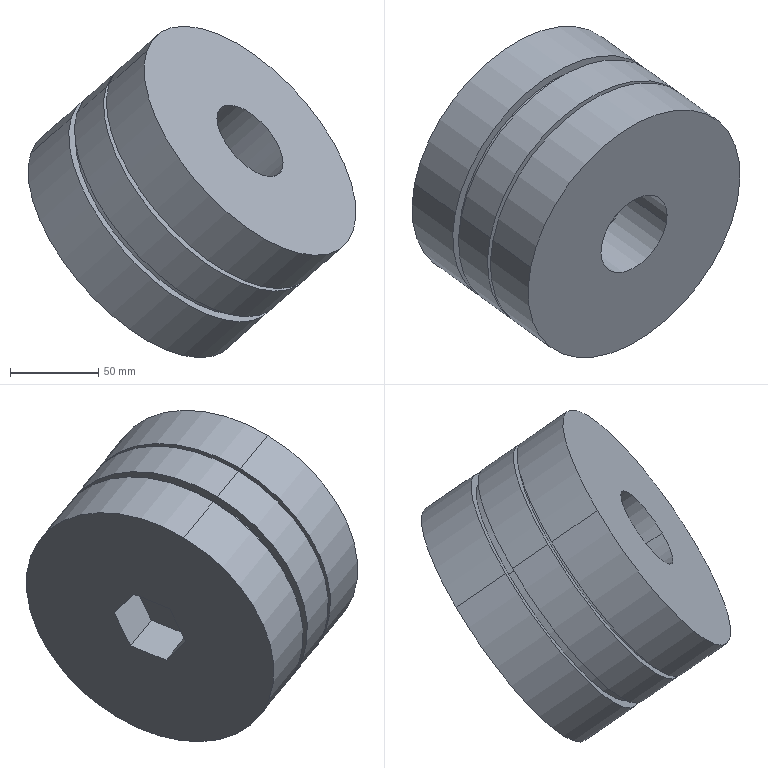Component | SolidWorks | FrictionWasher-1 | 1 solid | 29 faces | box 186.23 x 188.32 x 188.31 mm | volume 1876724 mm3 | plane 15 | cylinder 14 | commonest cylinder face diameters 160 x6 150 x4 50 x2 25 x2 | material Copper
STEP:
#1=CARTESIAN_POINT('',(0.3939,-67.745,7.065));
#2=VERTEX_POINT('',#1);
#3=CARTESIAN_POINT('',(-4.23,-69.254,11.068));
#4=VERTEX_POINT('',#3);
#5=CARTESIAN_POINT('',(-1.918,-68.5,9.067));
#6=DIRECTION('',(0.6592,-0.4763,0.5818));
#7=DIRECTION('',(0.734,0.2396,-0.6355));
#8=AXIS2_PLACEMENT_3D('',#5,#6,#7);
#9=CIRCLE('',#8,3.15);
#10=EDGE_CURVE('',#2,#4,#9,.T.);
#11=ORIENTED_EDGE('',*,*,#10,.F.);
#12=CARTESIAN_POINT('',(-0.4496,-67.136,6.321));
#13=VERTEX_POINT('',#12);
#14=CARTESIAN_POINT('',(0.3939,-67.745,7.065));
#15=DIRECTION('',(-0.6592,0.4763,-0.5818));
#16=VECTOR('',#15,39.37);
#17=LINE('',#14,#16);
#18=EDGE_CURVE('',#2,#13,#17,.T.);
#19=ORIENTED_EDGE('',*,*,#18,.T.);
#20=CARTESIAN_POINT('',(-5.073,-68.645,10.324));
#21=VERTEX_POINT('',#20);
#22=CARTESIAN_POINT('',(-2.761,-67.89,8.322));
#23=DIRECTION('',(-0.6592,0.4763,-0.5818));
#24=DIRECTION('',(-0.734,-0.2396,0.6355));
#25=AXIS2_PLACEMENT_3D('',#22,#23,#24);
#26=CIRCLE('',#25,3.15);
#27=EDGE_CURVE('',#21,#13,#26,.T.);
#28=ORIENTED_EDGE('',*,*,#27,.F.);
#29=CARTESIAN_POINT('',(-4.23,-69.254,11.068));
#30=DIRECTION('',(-0.6592,0.4763,-0.5818));
#31=VECTOR('',#30,39.37);
#32=LINE('',#29,#31);
#33=EDGE_CURVE('',#4,#21,#32,.T.);
#34=ORIENTED_EDGE('',*,*,#33,.F.);
#35=EDGE_LOOP('',(#11,#19,#28,#34));
#36=FACE_OUTER_BOUND('',#35,.T.);
#37=CARTESIAN_POINT('',(-1.918,-68.5,9.067));
#38=DIRECTION('',(-0.6592,0.4763,-0.5818));
#39=DIRECTION('',(-0.734,-0.2396,0.6355));
#40=AXIS2_PLACEMENT_3D('',#37,#38,#39);
#41=CYLINDRICAL_SURFACE('',#40,3.15);
#42=ADVANCED_FACE('',(#36),#41,.T.);
#43=CARTESIAN_POINT('',(-2.64,-68.736,9.692));
#44=VERTEX_POINT('',#43);
#45=CARTESIAN_POINT('',(-1.195,-68.264,8.441));
#46=VERTEX_POINT('',#45);
#47=CARTESIAN_POINT('',(-1.918,-68.5,9.067));
#48=DIRECTION('',(0.6592,-0.4763,0.5818));
#49=DIRECTION('',(0.734,0.2396,-0.6355));
#50=AXIS2_PLACEMENT_3D('',#47,#48,#49);
#51=CIRCLE('',#50,0.9843);
#52=EDGE_CURVE('',#44,#46,#51,.T.);
#53=ORIENTED_EDGE('',*,*,#52,.T.);
#54=CARTESIAN_POINT('',(-2.104,-67.608,7.64));
#55=VERTEX_POINT('',#54);
#56=CARTESIAN_POINT('',(-1.195,-68.264,8.441));
#57=DIRECTION('',(-0.6592,0.4763,-0.5818));
#58=VECTOR('',#57,39.37);
#59=LINE('',#56,#58);
#60=EDGE_CURVE('',#46,#55,#59,.T.);
#61=ORIENTED_EDGE('',*,*,#60,.T.);
#62=CARTESIAN_POINT('',(-3.549,-68.079,8.891));
#63=VERTEX_POINT('',#62);
#64=CARTESIAN_POINT('',(-2.826,-67.843,8.265));
#65=DIRECTION('',(0.6592,-0.4763,0.5818));
#66=DIRECTION('',(0.734,0.2396,-0.6355));
#67=AXIS2_PLACEMENT_3D('',#64,#65,#66);
#68=CIRCLE('',#67,0.9843);
#69=EDGE_CURVE('',#63,#55,#68,.T.);
#70=ORIENTED_EDGE('',*,*,#69,.F.);
#71=CARTESIAN_POINT('',(-2.64,-68.736,9.692));
#72=DIRECTION('',(-0.6592,0.4763,-0.5818));
#73=VECTOR('',#72,39.37);
#74=LINE('',#71,#73);
#75=EDGE_CURVE('',#44,#63,#74,.T.);
#76=ORIENTED_EDGE('',*,*,#75,.F.);
#77=EDGE_LOOP('',(#53,#61,#70,#76));
#78=FACE_OUTER_BOUND('',#77,.T.);
#79=CARTESIAN_POINT('',(-1.918,-68.5,9.067));
#80=DIRECTION('',(-0.6592,0.4763,-0.5818));
#81=DIRECTION('',(-0.734,-0.2396,0.6355));
#82=AXIS2_PLACEMENT_3D('',#79,#80,#81);
#83=CYLINDRICAL_SURFACE('',#82,0.9843);
#84=ADVANCED_FACE('',(#78),#83,.F.);
#85=CARTESIAN_POINT('',(-3.187,-67.961,8.578));
#86=VERTEX_POINT('',#85);
#87=CARTESIAN_POINT('',(-2.465,-67.726,7.952));
#88=VERTEX_POINT('',#87);
#89=CARTESIAN_POINT('',(-2.826,-67.843,8.265));
#90=DIRECTION('',(0.6592,-0.4763,0.5818));
#91=DIRECTION('',(0.734,0.2396,-0.6355));
#92=AXIS2_PLACEMENT_3D('',#89,#90,#91);
#93=CIRCLE('',#92,0.4921);
#94=EDGE_CURVE('',#86,#88,#93,.T.);
#95=ORIENTED_EDGE('',*,*,#94,.T.);
#96=CARTESIAN_POINT('',(-3.114,-67.257,7.38));
#97=VERTEX_POINT('',#96);
#98=CARTESIAN_POINT('',(-2.465,-67.726,7.952));
#99=DIRECTION('',(-0.6592,0.4763,-0.5818));
#100=VECTOR('',#99,39.37);
#101=LINE('',#98,#100);
#102=EDGE_CURVE('',#88,#97,#101,.T.);
#103=ORIENTED_EDGE('',*,*,#102,.T.);
#104=CARTESIAN_POINT('',(-3.836,-67.493,8.005));
#105=VERTEX_POINT('',#104);
#106=CARTESIAN_POINT('',(-3.475,-67.375,7.692));
#107=DIRECTION('',(0.6592,-0.4763,0.5818));
#108=DIRECTION('',(0.734,0.2396,-0.6355));
#109=AXIS2_PLACEMENT_3D('',#106,#107,#108);
#110=CIRCLE('',#109,0.4921);
#111=EDGE_CURVE('',#105,#97,#110,.T.);
#112=ORIENTED_EDGE('',*,*,#111,.F.);
#113=CARTESIAN_POINT('',(-3.187,-67.961,8.578));
#114=DIRECTION('',(-0.6592,0.4763,-0.5818));
#115=VECTOR('',#114,39.37);
#116=LINE('',#113,#115);
#117=EDGE_CURVE('',#86,#105,#116,.T.);
#118=ORIENTED_EDGE('',*,*,#117,.F.);
#119=EDGE_LOOP('',(#95,#103,#112,#118));
#120=FACE_OUTER_BOUND('',#119,.T.);
#121=CARTESIAN_POINT('',(-2.826,-67.843,8.265));
#122=DIRECTION('',(-0.6592,0.4763,-0.5818));
#123=DIRECTION('',(-0.734,-0.2396,0.6355));
#124=AXIS2_PLACEMENT_3D('',#121,#122,#123);
#125=CYLINDRICAL_SURFACE('',#124,0.4921);
#126=ADVANCED_FACE('',(#120),#125,.F.);
#127=CARTESIAN_POINT('',(-4.929,-68.598,10.199));
#128=VERTEX_POINT('',#127);
#129=CARTESIAN_POINT('',(-0.5941,-67.183,6.446));
#130=VERTEX_POINT('',#129);
#131=CARTESIAN_POINT('',(-2.761,-67.89,8.322));
#132=DIRECTION('',(-0.6592,0.4763,-0.5818));
#133=DIRECTION('',(-0.1633,-0.846,-0.5075));
#134=AXIS2_PLACEMENT_3D('',#131,#132,#133);
#135=CIRCLE('',#134,2.953);
#136=EDGE_CURVE('',#128,#130,#135,.T.);
#137=ORIENTED_EDGE('',*,*,#136,.T.);
#138=CARTESIAN_POINT('',(-0.659,-67.136,6.389));
#139=VERTEX_POINT('',#138);
#140=CARTESIAN_POINT('',(-0.5941,-67.183,6.446));
#141=DIRECTION('',(-0.6592,0.4763,-0.5818));
#142=VECTOR('',#141,39.37);
#143=LINE('',#140,#142);
#144=EDGE_CURVE('',#130,#139,#143,.T.);
#145=ORIENTED_EDGE('',*,*,#144,.T.);
#146=CARTESIAN_POINT('',(-4.994,-68.551,10.142));
#147=VERTEX_POINT('',#146);
#148=CARTESIAN_POINT('',(-2.826,-67.843,8.265));
#149=DIRECTION('',(-0.6592,0.4763,-0.5818));
#150=DIRECTION('',(-0.1633,-0.846,-0.5075));
#151=AXIS2_PLACEMENT_3D('',#148,#149,#150);
#152=CIRCLE('',#151,2.953);
#153=EDGE_CURVE('',#147,#139,#152,.T.);
#154=ORIENTED_EDGE('',*,*,#153,.F.);
#155=CARTESIAN_POINT('',(-4.929,-68.598,10.199));
#156=DIRECTION('',(-0.6592,0.4763,-0.5818));
#157=VECTOR('',#156,39.37);
#158=LINE('',#155,#157);
#159=EDGE_CURVE('',#128,#147,#158,.T.);
#160=ORIENTED_EDGE('',*,*,#159,.F.);
#161=EDGE_LOOP('',(#137,#145,#154,#160));
#162=FACE_OUTER_BOUND('',#161,.T.);
#163=CARTESIAN_POINT('',(-2.761,-67.89,8.322));
#164=DIRECTION('',(-0.6592,0.4763,-0.5818));
#165=DIRECTION('',(-0.734,-0.2396,0.6355));
#166=AXIS2_PLACEMENT_3D('',#163,#164,#165);
#167=CYLINDRICAL_SURFACE('',#166,2.953);
#168=ADVANCED_FACE('',(#162),#167,.T.);
#169=CARTESIAN_POINT('',(-5.917,-68.035,9.58));
#170=VERTEX_POINT('',#169);
#171=CARTESIAN_POINT('',(-1.293,-66.526,5.576));
#172=VERTEX_POINT('',#171);
#173=CARTESIAN_POINT('',(-3.605,-67.281,7.578));
#174=DIRECTION('',(-0.6592,0.4763,-0.5818));
#175=DIRECTION('',(-0.734,-0.2396,0.6355));
#176=AXIS2_PLACEMENT_3D('',#173,#174,#175);
#177=CIRCLE('',#176,3.15);
#178=EDGE_CURVE('',#170,#172,#177,.T.);
#179=ORIENTED_EDGE('',*,*,#178,.T.);
#180=CARTESIAN_POINT('',(-2.201,-65.87,4.775));
#181=VERTEX_POINT('',#180);
#182=CARTESIAN_POINT('',(0.3939,-67.745,7.065));
#183=DIRECTION('',(-0.6592,0.4763,-0.5818));
#184=VECTOR('',#183,39.37);
#185=LINE('',#182,#184);
#186=EDGE_CURVE('',#172,#181,#185,.T.);
#187=ORIENTED_EDGE('',*,*,#186,.T.);
#188=CARTESIAN_POINT('',(-6.825,-67.379,8.778));
#189=VERTEX_POINT('',#188);
#190=CARTESIAN_POINT('',(-4.513,-66.625,6.776));
#191=DIRECTION('',(0.6592,-0.4763,0.5818));
#192=DIRECTION('',(0.734,0.2396,-0.6355));
#193=AXIS2_PLACEMENT_3D('',#190,#191,#192);
#194=CIRCLE('',#193,3.15);
#195=EDGE_CURVE('',#181,#189,#194,.T.);
#196=ORIENTED_EDGE('',*,*,#195,.T.);
#197=CARTESIAN_POINT('',(-4.23,-69.254,11.068));
#198=DIRECTION('',(-0.6592,0.4763,-0.5818));
#199=VECTOR('',#198,39.37);
#200=LINE('',#197,#199);
#201=EDGE_CURVE('',#170,#189,#200,.T.);
#202=ORIENTED_EDGE('',*,*,#201,.F.);
#203=EDGE_LOOP('',(#179,#187,#196,#202));
#204=FACE_OUTER_BOUND('',#203,.T.);
#205=CARTESIAN_POINT('',(-1.918,-68.5,9.067));
#206=DIRECTION('',(-0.6592,0.4763,-0.5818));
#207=DIRECTION('',(-0.734,-0.2396,0.6355));
#208=AXIS2_PLACEMENT_3D('',#205,#206,#207);
#209=CYLINDRICAL_SURFACE('',#208,3.15);
#210=ADVANCED_FACE('',(#204),#209,.T.);
#211=CARTESIAN_POINT('',(-5.642,-68.082,9.569));
#212=VERTEX_POINT('',#211);
#213=CARTESIAN_POINT('',(-1.308,-66.667,5.816));
#214=VERTEX_POINT('',#213);
#215=CARTESIAN_POINT('',(-3.475,-67.375,7.692));
#216=DIRECTION('',(-0.6592,0.4763,-0.5818));
#217=DIRECTION('',(-0.1633,-0.846,-0.5075));
#218=AXIS2_PLACEMENT_3D('',#215,#216,#217);
#219=CIRCLE('',#218,2.953);
#220=EDGE_CURVE('',#212,#214,#219,.T.);
#221=ORIENTED_EDGE('',*,*,#220,.T.);
#222=CARTESIAN_POINT('',(-1.438,-66.574,5.701));
#223=VERTEX_POINT('',#222);
#224=CARTESIAN_POINT('',(-1.308,-66.667,5.816));
#225=DIRECTION('',(-0.6592,0.4763,-0.5818));
#226=VECTOR('',#225,39.37);
#227=LINE('',#224,#226);
#228=EDGE_CURVE('',#214,#223,#227,.T.);
#229=ORIENTED_EDGE('',*,*,#228,.T.);
#230=CARTESIAN_POINT('',(-5.772,-67.988,9.454));
#231=VERTEX_POINT('',#230);
#232=CARTESIAN_POINT('',(-3.605,-67.281,7.578));
#233=DIRECTION('',(-0.6592,0.4763,-0.5818));
#234=DIRECTION('',(-0.1633,-0.846,-0.5075));
#235=AXIS2_PLACEMENT_3D('',#232,#233,#234);
#236=CIRCLE('',#235,2.953);
#237=EDGE_CURVE('',#231,#223,#236,.T.);
#238=ORIENTED_EDGE('',*,*,#237,.F.);
#239=CARTESIAN_POINT('',(-5.642,-68.082,9.569));
#240=DIRECTION('',(-0.6592,0.4763,-0.5818));
#241=VECTOR('',#240,39.37);
#242=LINE('',#239,#241);
#243=EDGE_CURVE('',#212,#231,#242,.T.);
#244=ORIENTED_EDGE('',*,*,#243,.F.);
#245=EDGE_LOOP('',(#221,#229,#238,#244));
#246=FACE_OUTER_BOUND('',#245,.T.);
#247=CARTESIAN_POINT('',(-3.475,-67.375,7.692));
#248=DIRECTION('',(-0.6592,0.4763,-0.5818));
#249=DIRECTION('',(-0.734,-0.2396,0.6355));
#250=AXIS2_PLACEMENT_3D('',#247,#248,#249);
#251=CYLINDRICAL_SURFACE('',#250,2.953);
#252=ADVANCED_FACE('',(#246),#251,.T.);
#253=CARTESIAN_POINT('',(-5.138,-68.598,10.267));
#254=VERTEX_POINT('',#253);
#255=CARTESIAN_POINT('',(-0.5145,-67.089,6.264));
#256=VERTEX_POINT('',#255);
#257=CARTESIAN_POINT('',(-2.826,-67.843,8.265));
#258=DIRECTION('',(-0.6592,0.4763,-0.5818));
#259=DIRECTION('',(-0.734,-0.2396,0.6355));
#260=AXIS2_PLACEMENT_3D('',#257,#258,#259);
#261=CIRCLE('',#260,3.15);
#262=EDGE_CURVE('',#254,#256,#261,.T.);
#263=ORIENTED_EDGE('',*,*,#262,.T.);
#264=CARTESIAN_POINT('',(-1.163,-66.62,5.691));
#265=VERTEX_POINT('',#264);
#266=CARTESIAN_POINT('',(0.3939,-67.745,7.065));
#267=DIRECTION('',(-0.6592,0.4763,-0.5818));
#268=VECTOR('',#267,39.37);
#269=LINE('',#266,#268);
#270=EDGE_CURVE('',#256,#265,#269,.T.);
#271=ORIENTED_EDGE('',*,*,#270,.T.);
#272=CARTESIAN_POINT('',(-5.787,-68.129,9.694));
#273=VERTEX_POINT('',#272);
#274=CARTESIAN_POINT('',(-3.475,-67.375,7.692));
#275=DIRECTION('',(-0.6592,0.4763,-0.5818));
#276=DIRECTION('',(-0.734,-0.2396,0.6355));
#277=AXIS2_PLACEMENT_3D('',#274,#275,#276);
#278=CIRCLE('',#277,3.15);
#279=EDGE_CURVE('',#273,#265,#278,.T.);
#280=ORIENTED_EDGE('',*,*,#279,.F.);
#281=CARTESIAN_POINT('',(-4.23,-69.254,11.068));
#282=DIRECTION('',(-0.6592,0.4763,-0.5818));
#283=VECTOR('',#282,39.37);
#284=LINE('',#281,#283);
#285=EDGE_CURVE('',#254,#273,#284,.T.);
#286=ORIENTED_EDGE('',*,*,#285,.F.);
#287=EDGE_LOOP('',(#263,#271,#280,#286));
#288=FACE_OUTER_BOUND('',#287,.T.);
#289=CARTESIAN_POINT('',(-1.918,-68.5,9.067));
#290=DIRECTION('',(-0.6592,0.4763,-0.5818));
#291=DIRECTION('',(-0.734,-0.2396,0.6355));
#292=AXIS2_PLACEMENT_3D('',#289,#290,#291);
#293=CYLINDRICAL_SURFACE('',#292,3.15);
#294=ADVANCED_FACE('',(#288),#293,.T.);
#295=ORIENTED_EDGE('',*,*,#270,.F.);
#296=CARTESIAN_POINT('',(-2.826,-67.843,8.265));
#297=DIRECTION('',(-0.6592,0.4763,-0.5818));
#298=DIRECTION('',(-0.734,-0.2396,0.6355));
#299=AXIS2_PLACEMENT_3D('',#296,#297,#298);
#300=CIRCLE('',#299,3.15);
#301=EDGE_CURVE('',#256,#254,#300,.T.);
#302=ORIENTED_EDGE('',*,*,#301,.T.);
#303=ORIENTED_EDGE('',*,*,#285,.T.);
#304=CARTESIAN_POINT('',(-3.475,-67.375,7.692));
#305=DIRECTION('',(-0.6592,0.4763,-0.5818));
#306=DIRECTION('',(-0.734,-0.2396,0.6355));
#307=AXIS2_PLACEMENT_3D('',#304,#305,#306);
#308=CIRCLE('',#307,3.15);
#309=EDGE_CURVE('',#265,#273,#308,.T.);
#310=ORIENTED_EDGE('',*,*,#309,.F.);
#311=EDGE_LOOP('',(#295,#302,#303,#310));
#312=FACE_OUTER_BOUND('',#311,.T.);
#313=CARTESIAN_POINT('',(-1.918,-68.5,9.067));
#314=DIRECTION('',(-0.6592,0.4763,-0.5818));
#315=DIRECTION('',(-0.734,-0.2396,0.6355));
#316=AXIS2_PLACEMENT_3D('',#313,#314,#315);
#317=CYLINDRICAL_SURFACE('',#316,3.15);
#318=ADVANCED_FACE('',(#312),#317,.T.);
#319=ORIENTED_EDGE('',*,*,#220,.F.);
#320=CARTESIAN_POINT('',(-3.475,-67.375,7.692));
#321=DIRECTION('',(-0.6592,0.4763,-0.5818));
#322=DIRECTION('',(-0.1633,-0.846,-0.5075));
#323=AXIS2_PLACEMENT_3D('',#320,#321,#322);
#324=CIRCLE('',#323,2.953);
#325=EDGE_CURVE('',#214,#212,#324,.T.);
#326=ORIENTED_EDGE('',*,*,#325,.F.);
#327=EDGE_LOOP('',(#319,#326));
#328=FACE_BOUND('',#327,.T.);
#329=ORIENTED_EDGE('',*,*,#279,.T.);
#330=ORIENTED_EDGE('',*,*,#309,.T.);
#331=EDGE_LOOP('',(#329,#330));
#332=FACE_OUTER_BOUND('',#331,.T.);
#333=CARTESIAN_POINT('',(-3.475,-67.375,7.692));
#334=DIRECTION('',(-0.6592,0.4763,-0.5818));
#335=DIRECTION('',(-0.734,-0.2396,0.6355));
#336=AXIS2_PLACEMENT_3D('',#333,#334,#335);
#337=PLANE('',#336);
#338=ADVANCED_FACE('',(#328,#332),#337,.T.);
#339=ORIENTED_EDGE('',*,*,#237,.T.);
#340=CARTESIAN_POINT('',(-3.605,-67.281,7.578));
#341=DIRECTION('',(-0.6592,0.4763,-0.5818));
#342=DIRECTION('',(-0.1633,-0.846,-0.5075));
#343=AXIS2_PLACEMENT_3D('',#340,#341,#342);
#344=CIRCLE('',#343,2.953);
#345=EDGE_CURVE('',#223,#231,#344,.T.);
#346=ORIENTED_EDGE('',*,*,#345,.T.);
#347=EDGE_LOOP('',(#339,#346));
#348=FACE_BOUND('',#347,.T.);
#349=ORIENTED_EDGE('',*,*,#178,.F.);
#350=CARTESIAN_POINT('',(-3.605,-67.281,7.578));
#351=DIRECTION('',(-0.6592,0.4763,-0.5818));
#352=DIRECTION('',(-0.734,-0.2396,0.6355));
#353=AXIS2_PLACEMENT_3D('',#350,#351,#352);
#354=CIRCLE('',#353,3.15);
#355=EDGE_CURVE('',#172,#170,#354,.T.);
#356=ORIENTED_EDGE('',*,*,#355,.F.);
#357=EDGE_LOOP('',(#349,#356));
#358=FACE_OUTER_BOUND('',#357,.T.);
#359=CARTESIAN_POINT('',(-3.605,-67.281,7.578));
#360=DIRECTION('',(-0.6592,0.4763,-0.5818));
#361=DIRECTION('',(-0.734,-0.2396,0.6355));
#362=AXIS2_PLACEMENT_3D('',#359,#360,#361);
#363=PLANE('',#362);
#364=ADVANCED_FACE('',(#348,#358),#363,.F.);
#365=ORIENTED_EDGE('',*,*,#228,.F.);
#366=ORIENTED_EDGE('',*,*,#325,.T.);
#367=ORIENTED_EDGE('',*,*,#243,.T.);
#368=ORIENTED_EDGE('',*,*,#345,.F.);
#369=EDGE_LOOP('',(#365,#366,#367,#368));
#370=FACE_OUTER_BOUND('',#369,.T.);
#371=CARTESIAN_POINT('',(-3.475,-67.375,7.692));
#372=DIRECTION('',(-0.6592,0.4763,-0.5818));
#373=DIRECTION('',(-0.734,-0.2396,0.6355));
#374=AXIS2_PLACEMENT_3D('',#371,#372,#373);
#375=CYLINDRICAL_SURFACE('',#374,2.953);
#376=ADVANCED_FACE('',(#370),#375,.T.);
#377=CARTESIAN_POINT('',(-3.183,-66.656,6.935));
#378=VERTEX_POINT('',#377);
#379=CARTESIAN_POINT('',(-3.474,-67.454,6.611));
#380=VERTEX_POINT('',#379);
#381=CARTESIAN_POINT('',(-3.183,-66.656,6.935));
#382=DIRECTION('',(-0.3203,-0.8779,-0.3559));
#383=VECTOR('',#382,39.37);
#384=LINE('',#381,#383);
#385=EDGE_CURVE('',#378,#380,#384,.T.);
#386=ORIENTED_EDGE('',*,*,#385,.T.);
#387=CARTESIAN_POINT('',(-4.156,-67.892,7.025));
#388=VERTEX_POINT('',#387);
#389=CARTESIAN_POINT('',(-3.474,-67.454,6.611));
#390=DIRECTION('',(-0.7493,-0.4808,0.4554));
#391=VECTOR('',#390,39.37);
#392=LINE('',#389,#391);
#393=EDGE_CURVE('',#380,#388,#392,.T.);
#394=ORIENTED_EDGE('',*,*,#393,.T.);
#395=CARTESIAN_POINT('',(-4.546,-67.53,7.763));
#396=VERTEX_POINT('',#395);
#397=CARTESIAN_POINT('',(-4.156,-67.892,7.025));
#398=DIRECTION('',(-0.4291,0.3972,0.8113));
#399=VECTOR('',#398,39.37);
#400=LINE('',#397,#399);
#401=EDGE_CURVE('',#388,#396,#400,.T.);
#402=ORIENTED_EDGE('',*,*,#401,.T.);
#403=CARTESIAN_POINT('',(-4.255,-66.732,8.086));
#404=VERTEX_POINT('',#403);
#405=CARTESIAN_POINT('',(-4.546,-67.53,7.763));
#406=DIRECTION('',(0.3203,0.8779,0.3559));
#407=VECTOR('',#406,39.37);
#408=LINE('',#405,#407);
#409=EDGE_CURVE('',#396,#404,#408,.T.);
#410=ORIENTED_EDGE('',*,*,#409,.T.);
#411=CARTESIAN_POINT('',(-3.573,-66.295,7.672));
#412=VERTEX_POINT('',#411);
#413=CARTESIAN_POINT('',(-4.255,-66.732,8.086));
#414=DIRECTION('',(0.7493,0.4808,-0.4554));
#415=VECTOR('',#414,39.37);
#416=LINE('',#413,#415);
#417=EDGE_CURVE('',#404,#412,#416,.T.);
#418=ORIENTED_EDGE('',*,*,#417,.T.);
#419=CARTESIAN_POINT('',(-3.573,-66.295,7.672));
#420=DIRECTION('',(0.4291,-0.3972,-0.8113));
#421=VECTOR('',#420,39.37);
#422=LINE('',#419,#421);
#423=EDGE_CURVE('',#412,#378,#422,.T.);
#424=ORIENTED_EDGE('',*,*,#423,.T.);
#425=EDGE_LOOP('',(#386,#394,#402,#410,#418,#424));
#426=FACE_OUTER_BOUND('',#425,.T.);
#427=CARTESIAN_POINT('',(-3.864,-67.093,7.349));
#428=DIRECTION('',(-0.6592,0.4763,-0.5818));
#429=DIRECTION('',(-0.734,-0.2396,0.6355));
#430=AXIS2_PLACEMENT_3D('',#427,#428,#429);
#431=PLANE('',#430);
#432=ADVANCED_FACE('',(#426),#431,.T.);
#433=CARTESIAN_POINT('',(-4.804,-67.423,6.453));
#434=VERTEX_POINT('',#433);
#435=CARTESIAN_POINT('',(-5.195,-67.062,7.19));
#436=VERTEX_POINT('',#435);
#437=CARTESIAN_POINT('',(-4.804,-67.423,6.453));
#438=DIRECTION('',(-0.4291,0.3972,0.8113));
#439=VECTOR('',#438,39.37);
#440=LINE('',#437,#439);
#441=EDGE_CURVE('',#434,#436,#440,.T.);
#442=ORIENTED_EDGE('',*,*,#441,.T.);
#443=CARTESIAN_POINT('',(-4.546,-67.53,7.763));
#444=DIRECTION('',(-0.6592,0.4763,-0.5818));
#445=VECTOR('',#444,39.37);
#446=LINE('',#443,#445);
#447=EDGE_CURVE('',#396,#436,#446,.T.);
#448=ORIENTED_EDGE('',*,*,#447,.F.);
#449=ORIENTED_EDGE('',*,*,#401,.F.);
#450=CARTESIAN_POINT('',(-4.156,-67.892,7.025));
#451=DIRECTION('',(-0.6592,0.4763,-0.5818));
#452=VECTOR('',#451,39.37);
#453=LINE('',#450,#452);
#454=EDGE_CURVE('',#388,#434,#453,.T.);
#455=ORIENTED_EDGE('',*,*,#454,.T.);
#456=EDGE_LOOP('',(#442,#448,#449,#455));
#457=FACE_OUTER_BOUND('',#456,.T.);
#458=CARTESIAN_POINT('',(-4.156,-67.892,7.025));
#459=DIRECTION('',(-0.6175,-0.7844,0.05746));
#460=DIRECTION('',(0.4291,-0.3972,-0.8113));
#461=AXIS2_PLACEMENT_3D('',#458,#459,#460);
#462=PLANE('',#461);
#463=ADVANCED_FACE('',(#457),#462,.F.);
#464=CARTESIAN_POINT('',(-4.903,-66.263,7.514));
#465=VERTEX_POINT('',#464);
#466=CARTESIAN_POINT('',(-5.195,-67.062,7.19));
#467=DIRECTION('',(0.3203,0.8779,0.3559));
#468=VECTOR('',#467,39.37);
#469=LINE('',#466,#468);
#470=EDGE_CURVE('',#436,#465,#469,.T.);
#471=ORIENTED_EDGE('',*,*,#470,.T.);
#472=CARTESIAN_POINT('',(-4.255,-66.732,8.086));
#473=DIRECTION('',(-0.6592,0.4763,-0.5818));
#474=VECTOR('',#473,39.37);
#475=LINE('',#472,#474);
#476=EDGE_CURVE('',#404,#465,#475,.T.);
#477=ORIENTED_EDGE('',*,*,#476,.F.);
#478=ORIENTED_EDGE('',*,*,#409,.F.);
#479=ORIENTED_EDGE('',*,*,#447,.T.);
#480=EDGE_LOOP('',(#471,#477,#478,#479));
#481=FACE_OUTER_BOUND('',#480,.T.);
#482=CARTESIAN_POINT('',(-4.546,-67.53,7.763));
#483=DIRECTION('',(-0.6803,-0.04826,0.7313));
#484=DIRECTION('',(-0.3203,-0.8779,-0.3559));
#485=AXIS2_PLACEMENT_3D('',#482,#483,#484);
#486=PLANE('',#485);
#487=ADVANCED_FACE('',(#481),#486,.F.);
#488=CARTESIAN_POINT('',(-4.222,-65.826,7.1));
#489=VERTEX_POINT('',#488);
#490=CARTESIAN_POINT('',(-4.903,-66.263,7.514));
#491=DIRECTION('',(0.7493,0.4808,-0.4554));
#492=VECTOR('',#491,39.37);
#493=LINE('',#490,#492);
#494=EDGE_CURVE('',#465,#489,#493,.T.);
#495=ORIENTED_EDGE('',*,*,#494,.T.);
#496=CARTESIAN_POINT('',(-3.573,-66.295,7.672));
#497=DIRECTION('',(-0.6592,0.4763,-0.5818));
#498=VECTOR('',#497,39.37);
#499=LINE('',#496,#498);
#500=EDGE_CURVE('',#412,#489,#499,.T.);
#501=ORIENTED_EDGE('',*,*,#500,.F.);
#502=ORIENTED_EDGE('',*,*,#417,.F.);
#503=ORIENTED_EDGE('',*,*,#476,.T.);
#504=EDGE_LOOP('',(#495,#501,#502,#503));
#505=FACE_OUTER_BOUND('',#504,.T.);
#506=CARTESIAN_POINT('',(-4.255,-66.732,8.086));
#507=DIRECTION('',(-0.0628,0.7362,0.6739));
#508=DIRECTION('',(-0.7493,-0.4808,0.4554));
#509=AXIS2_PLACEMENT_3D('',#506,#507,#508);
#510=PLANE('',#509);
#511=ADVANCED_FACE('',(#505),#510,.F.);
#512=CARTESIAN_POINT('',(-3.832,-66.187,6.362));
#513=VERTEX_POINT('',#512);
#514=CARTESIAN_POINT('',(-4.222,-65.826,7.1));
#515=DIRECTION('',(0.4291,-0.3972,-0.8113));
#516=VECTOR('',#515,39.37);
#517=LINE('',#514,#516);
#518=EDGE_CURVE('',#489,#513,#517,.T.);
#519=ORIENTED_EDGE('',*,*,#518,.T.);
#520=CARTESIAN_POINT('',(-3.183,-66.656,6.935));
#521=DIRECTION('',(-0.6592,0.4763,-0.5818));
#522=VECTOR('',#521,39.37);
#523=LINE('',#520,#522);
#524=EDGE_CURVE('',#378,#513,#523,.T.);
#525=ORIENTED_EDGE('',*,*,#524,.F.);
#526=ORIENTED_EDGE('',*,*,#423,.F.);
#527=ORIENTED_EDGE('',*,*,#500,.T.);
#528=EDGE_LOOP('',(#519,#525,#526,#527));
#529=FACE_OUTER_BOUND('',#528,.T.);
#530=CARTESIAN_POINT('',(-3.573,-66.295,7.672));
#531=DIRECTION('',(0.6175,0.7844,-0.05746));
#532=DIRECTION('',(-0.4291,0.3972,0.8113));
#533=AXIS2_PLACEMENT_3D('',#530,#531,#532);
#534=PLANE('',#533);
#535=ADVANCED_FACE('',(#529),#534,.F.);
#536=CARTESIAN_POINT('',(-4.123,-66.986,6.039));
#537=VERTEX_POINT('',#536);
#538=CARTESIAN_POINT('',(-3.832,-66.187,6.362));
#539=DIRECTION('',(-0.3203,-0.8779,-0.3559));
#540=VECTOR('',#539,39.37);
#541=LINE('',#538,#540);
#542=EDGE_CURVE('',#513,#537,#541,.T.);
#543=ORIENTED_EDGE('',*,*,#542,.T.);
#544=CARTESIAN_POINT('',(-3.474,-67.454,6.611));
#545=DIRECTION('',(-0.6592,0.4763,-0.5818));
#546=VECTOR('',#545,39.37);
#547=LINE('',#544,#546);
#548=EDGE_CURVE('',#380,#537,#547,.T.);
#549=ORIENTED_EDGE('',*,*,#548,.F.);
#550=ORIENTED_EDGE('',*,*,#385,.F.);
#551=ORIENTED_EDGE('',*,*,#524,.T.);
#552=EDGE_LOOP('',(#543,#549,#550,#551));
#553=FACE_OUTER_BOUND('',#552,.T.);
#554=CARTESIAN_POINT('',(-3.183,-66.656,6.935));
#555=DIRECTION('',(0.6803,0.04826,-0.7313));
#556=DIRECTION('',(0.3203,0.8779,0.3559));
#557=AXIS2_PLACEMENT_3D('',#554,#555,#556);
#558=PLANE('',#557);
#559=ADVANCED_FACE('',(#553),#558,.F.);
#560=CARTESIAN_POINT('',(-4.123,-66.986,6.039));
#561=DIRECTION('',(-0.7493,-0.4808,0.4554));
#562=VECTOR('',#561,39.37);
#563=LINE('',#560,#562);
#564=EDGE_CURVE('',#537,#434,#563,.T.);
#565=ORIENTED_EDGE('',*,*,#564,.T.);
#566=ORIENTED_EDGE('',*,*,#454,.F.);
#567=ORIENTED_EDGE('',*,*,#393,.F.);
#568=ORIENTED_EDGE('',*,*,#548,.T.);
#569=EDGE_LOOP('',(#565,#566,#567,#568));
#570=FACE_OUTER_BOUND('',#569,.T.);
#571=CARTESIAN_POINT('',(-3.474,-67.454,6.611));
#572=DIRECTION('',(0.0628,-0.7362,-0.6739));
#573=DIRECTION('',(0.7493,0.4808,-0.4554));
#574=AXIS2_PLACEMENT_3D('',#571,#572,#573);
#575=PLANE('',#574);
#576=ADVANCED_FACE('',(#570),#575,.F.);
#577=ORIENTED_EDGE('',*,*,#564,.F.);
#578=ORIENTED_EDGE('',*,*,#542,.F.);
#579=ORIENTED_EDGE('',*,*,#518,.F.);
#580=ORIENTED_EDGE('',*,*,#494,.F.);
#581=ORIENTED_EDGE('',*,*,#470,.F.);
#582=ORIENTED_EDGE('',*,*,#441,.F.);
#583=EDGE_LOOP('',(#577,#578,#579,#580,#581,#582));
#584=FACE_BOUND('',#583,.T.);
#585=CARTESIAN_POINT('',(-4.513,-66.625,6.776));
#586=DIRECTION('',(0.6592,-0.4763,0.5818));
#587=DIRECTION('',(0.734,0.2396,-0.6355));
#588=AXIS2_PLACEMENT_3D('',#585,#586,#587);
#589=CIRCLE('',#588,3.15);
#590=EDGE_CURVE('',#189,#181,#589,.T.);
#591=ORIENTED_EDGE('',*,*,#590,.F.);
#592=ORIENTED_EDGE('',*,*,#195,.F.);
#593=EDGE_LOOP('',(#591,#592));
#594=FACE_OUTER_BOUND('',#593,.T.);
#595=CARTESIAN_POINT('',(-4.513,-66.625,6.776));
#596=DIRECTION('',(0.6592,-0.4763,0.5818));
#597=DIRECTION('',(0.734,0.2396,-0.6355));
#598=AXIS2_PLACEMENT_3D('',#595,#596,#597);
#599=PLANE('',#598);
#600=ADVANCED_FACE('',(#584,#594),#599,.F.);
#601=ORIENTED_EDGE('',*,*,#186,.F.);
#602=ORIENTED_EDGE('',*,*,#355,.T.);
#603=ORIENTED_EDGE('',*,*,#201,.T.);
#604=ORIENTED_EDGE('',*,*,#590,.T.);
#605=EDGE_LOOP('',(#601,#602,#603,#604));
#606=FACE_OUTER_BOUND('',#605,.T.);
#607=CARTESIAN_POINT('',(-1.918,-68.5,9.067));
#608=DIRECTION('',(-0.6592,0.4763,-0.5818));
#609=DIRECTION('',(-0.734,-0.2396,0.6355));
#610=AXIS2_PLACEMENT_3D('',#607,#608,#609);
#611=CYLINDRICAL_SURFACE('',#610,3.15);
#612=ADVANCED_FACE('',(#606),#611,.T.);
#613=ORIENTED_EDGE('',*,*,#136,.F.);
#614=CARTESIAN_POINT('',(-2.761,-67.89,8.322));
#615=DIRECTION('',(-0.6592,0.4763,-0.5818));
#616=DIRECTION('',(-0.1633,-0.846,-0.5075));
#617=AXIS2_PLACEMENT_3D('',#614,#615,#616);
#618=CIRCLE('',#617,2.953);
#619=EDGE_CURVE('',#130,#128,#618,.T.);
#620=ORIENTED_EDGE('',*,*,#619,.F.);
#621=EDGE_LOOP('',(#613,#620));
#622=FACE_BOUND('',#621,.T.);
#623=ORIENTED_EDGE('',*,*,#27,.T.);
#624=CARTESIAN_POINT('',(-2.761,-67.89,8.322));
#625=DIRECTION('',(-0.6592,0.4763,-0.5818));
#626=DIRECTION('',(-0.734,-0.2396,0.6355));
#627=AXIS2_PLACEMENT_3D('',#624,#625,#626);
#628=CIRCLE('',#627,3.15);
#629=EDGE_CURVE('',#13,#21,#628,.T.);
#630=ORIENTED_EDGE('',*,*,#629,.T.);
#631=EDGE_LOOP('',(#623,#630));
#632=FACE_OUTER_BOUND('',#631,.T.);
#633=CARTESIAN_POINT('',(-2.761,-67.89,8.322));
#634=DIRECTION('',(-0.6592,0.4763,-0.5818));
#635=DIRECTION('',(-0.734,-0.2396,0.6355));
#636=AXIS2_PLACEMENT_3D('',#633,#634,#635);
#637=PLANE('',#636);
#638=ADVANCED_FACE('',(#622,#632),#637,.T.);
#639=ORIENTED_EDGE('',*,*,#153,.T.);
#640=CARTESIAN_POINT('',(-2.826,-67.843,8.265));
#641=DIRECTION('',(-0.6592,0.4763,-0.5818));
#642=DIRECTION('',(-0.1633,-0.846,-0.5075));
#643=AXIS2_PLACEMENT_3D('',#640,#641,#642);
#644=CIRCLE('',#643,2.953);
#645=EDGE_CURVE('',#139,#147,#644,.T.);
#646=ORIENTED_EDGE('',*,*,#645,.T.);
#647=EDGE_LOOP('',(#639,#646));
#648=FACE_BOUND('',#647,.T.);
#649=ORIENTED_EDGE('',*,*,#262,.F.);
#650=ORIENTED_EDGE('',*,*,#301,.F.);
#651=EDGE_LOOP('',(#649,#650));
#652=FACE_OUTER_BOUND('',#651,.T.);
#653=CARTESIAN_POINT('',(-2.826,-67.843,8.265));
#654=DIRECTION('',(-0.6592,0.4763,-0.5818));
#655=DIRECTION('',(-0.734,-0.2396,0.6355));
#656=AXIS2_PLACEMENT_3D('',#653,#654,#655);
#657=PLANE('',#656);
#658=ADVANCED_FACE('',(#648,#652),#657,.F.);
#659=ORIENTED_EDGE('',*,*,#144,.F.);
#660=ORIENTED_EDGE('',*,*,#619,.T.);
#661=ORIENTED_EDGE('',*,*,#159,.T.);
#662=ORIENTED_EDGE('',*,*,#645,.F.);
#663=EDGE_LOOP('',(#659,#660,#661,#662));
#664=FACE_OUTER_BOUND('',#663,.T.);
#665=CARTESIAN_POINT('',(-2.761,-67.89,8.322));
#666=DIRECTION('',(-0.6592,0.4763,-0.5818));
#667=DIRECTION('',(-0.734,-0.2396,0.6355));
#668=AXIS2_PLACEMENT_3D('',#665,#666,#667);
#669=CYLINDRICAL_SURFACE('',#668,2.953);
#670=ADVANCED_FACE('',(#664),#669,.T.);
#671=ORIENTED_EDGE('',*,*,#111,.T.);
#672=CARTESIAN_POINT('',(-3.475,-67.375,7.692));
#673=DIRECTION('',(0.6592,-0.4763,0.5818));
#674=DIRECTION('',(0.734,0.2396,-0.6355));
#675=AXIS2_PLACEMENT_3D('',#672,#673,#674);
#676=CIRCLE('',#675,0.4921);
#677=EDGE_CURVE('',#97,#105,#676,.T.);
#678=ORIENTED_EDGE('',*,*,#677,.T.);
#679=EDGE_LOOP('',(#671,#678));
#680=FACE_OUTER_BOUND('',#679,.T.);
#681=CARTESIAN_POINT('',(-3.475,-67.375,7.692));
#682=DIRECTION('',(0.6592,-0.4763,0.5818));
#683=DIRECTION('',(0.734,0.2396,-0.6355));
#684=AXIS2_PLACEMENT_3D('',#681,#682,#683);
#685=PLANE('',#684);
#686=ADVANCED_FACE('',(#680),#685,.T.);
#687=ORIENTED_EDGE('',*,*,#102,.F.);
#688=CARTESIAN_POINT('',(-2.826,-67.843,8.265));
#689=DIRECTION('',(0.6592,-0.4763,0.5818));
#690=DIRECTION('',(0.734,0.2396,-0.6355));
#691=AXIS2_PLACEMENT_3D('',#688,#689,#690);
#692=CIRCLE('',#691,0.4921);
#693=EDGE_CURVE('',#88,#86,#692,.T.);
#694=ORIENTED_EDGE('',*,*,#693,.T.);
#695=ORIENTED_EDGE('',*,*,#117,.T.);
#696=ORIENTED_EDGE('',*,*,#677,.F.);
#697=EDGE_LOOP('',(#687,#694,#695,#696));
#698=FACE_OUTER_BOUND('',#697,.T.);
#699=CARTESIAN_POINT('',(-2.826,-67.843,8.265));
#700=DIRECTION('',(-0.6592,0.4763,-0.5818));
#701=DIRECTION('',(-0.734,-0.2396,0.6355));
#702=AXIS2_PLACEMENT_3D('',#699,#700,#701);
#703=CYLINDRICAL_SURFACE('',#702,0.4921);
#704=ADVANCED_FACE('',(#698),#703,.F.);
#705=ORIENTED_EDGE('',*,*,#94,.F.);
#706=ORIENTED_EDGE('',*,*,#693,.F.);
#707=EDGE_LOOP('',(#705,#706));
#708=FACE_BOUND('',#707,.T.);
#709=ORIENTED_EDGE('',*,*,#69,.T.);
#710=CARTESIAN_POINT('',(-2.826,-67.843,8.265));
#711=DIRECTION('',(0.6592,-0.4763,0.5818));
#712=DIRECTION('',(0.734,0.2396,-0.6355));
#713=AXIS2_PLACEMENT_3D('',#710,#711,#712);
#714=CIRCLE('',#713,0.9843);
#715=EDGE_CURVE('',#55,#63,#714,.T.);
#716=ORIENTED_EDGE('',*,*,#715,.T.);
#717=EDGE_LOOP('',(#709,#716));
#718=FACE_OUTER_BOUND('',#717,.T.);
#719=CARTESIAN_POINT('',(-2.826,-67.843,8.265));
#720=DIRECTION('',(0.6592,-0.4763,0.5818));
#721=DIRECTION('',(0.734,0.2396,-0.6355));
#722=AXIS2_PLACEMENT_3D('',#719,#720,#721);
#723=PLANE('',#722);
#724=ADVANCED_FACE('',(#708,#718),#723,.T.);
#725=ORIENTED_EDGE('',*,*,#60,.F.);
#726=CARTESIAN_POINT('',(-1.918,-68.5,9.067));
#727=DIRECTION('',(0.6592,-0.4763,0.5818));
#728=DIRECTION('',(0.734,0.2396,-0.6355));
#729=AXIS2_PLACEMENT_3D('',#726,#727,#728);
#730=CIRCLE('',#729,0.9843);
#731=EDGE_CURVE('',#46,#44,#730,.T.);
#732=ORIENTED_EDGE('',*,*,#731,.T.);
#733=ORIENTED_EDGE('',*,*,#75,.T.);
#734=ORIENTED_EDGE('',*,*,#715,.F.);
#735=EDGE_LOOP('',(#725,#732,#733,#734));
#736=FACE_OUTER_BOUND('',#735,.T.);
#737=CARTESIAN_POINT('',(-1.918,-68.5,9.067));
#738=DIRECTION('',(-0.6592,0.4763,-0.5818));
#739=DIRECTION('',(-0.734,-0.2396,0.6355));
#740=AXIS2_PLACEMENT_3D('',#737,#738,#739);
#741=CYLINDRICAL_SURFACE('',#740,0.9843);
#742=ADVANCED_FACE('',(#736),#741,.F.);
#743=ORIENTED_EDGE('',*,*,#52,.F.);
#744=ORIENTED_EDGE('',*,*,#731,.F.);
#745=EDGE_LOOP('',(#743,#744));
#746=FACE_BOUND('',#745,.T.);
#747=CARTESIAN_POINT('',(-1.918,-68.5,9.067));
#748=DIRECTION('',(0.6592,-0.4763,0.5818));
#749=DIRECTION('',(0.734,0.2396,-0.6355));
#750=AXIS2_PLACEMENT_3D('',#747,#748,#749);
#751=CIRCLE('',#750,3.15);
#752=EDGE_CURVE('',#4,#2,#751,.T.);
#753=ORIENTED_EDGE('',*,*,#752,.T.);
#754=ORIENTED_EDGE('',*,*,#10,.T.);
#755=EDGE_LOOP('',(#753,#754));
#756=FACE_OUTER_BOUND('',#755,.T.);
#757=CARTESIAN_POINT('',(-1.918,-68.5,9.067));
#758=DIRECTION('',(0.6592,-0.4763,0.5818));
#759=DIRECTION('',(0.734,0.2396,-0.6355));
#760=AXIS2_PLACEMENT_3D('',#757,#758,#759);
#761=PLANE('',#760);
#762=ADVANCED_FACE('',(#746,#756),#761,.T.);
#763=ORIENTED_EDGE('',*,*,#18,.F.);
#764=ORIENTED_EDGE('',*,*,#752,.F.);
#765=ORIENTED_EDGE('',*,*,#33,.T.);
#766=ORIENTED_EDGE('',*,*,#629,.F.);
#767=EDGE_LOOP('',(#763,#764,#765,#766));
#768=FACE_OUTER_BOUND('',#767,.T.);
#769=CARTESIAN_POINT('',(-1.918,-68.5,9.067));
#770=DIRECTION('',(-0.6592,0.4763,-0.5818));
#771=DIRECTION('',(-0.734,-0.2396,0.6355));
#772=AXIS2_PLACEMENT_3D('',#769,#770,#771);
#773=CYLINDRICAL_SURFACE('',#772,3.15);
#774=ADVANCED_FACE('',(#768),#773,.T.);
#775=CLOSED_SHELL('',(#42,#84,#126,#168,#210,#252,#294,#318,#338,#364,#376,#432,#463,#487,#511,#535,#559,#576,#600,#612,#638,#658,#670,#686,#704,#724,#742,#762,#774));
#776=MANIFOLD_SOLID_BREP('',#775);
#777=CARTESIAN_POINT('',(0.,0.,0.));
#778=DIRECTION('',(0.,0.,1.));
#779=DIRECTION('',(1.,0.,0.));
#780=AXIS2_PLACEMENT_3D('',#777,#778,#779);
#781=(LENGTH_UNIT()NAMED_UNIT(*)SI_UNIT($,.METRE.));
#782=LENGTH_MEASURE_WITH_UNIT(LENGTH_MEASURE(0.0254),#781);
#783=DIMENSIONAL_EXPONENTS(1.,0.,0.,0.,0.,0.,0.);
#784=(CONVERSION_BASED_UNIT('',#782)LENGTH_UNIT()NAMED_UNIT(#783));
#785=UNCERTAINTY_MEASURE_WITH_UNIT(LENGTH_MEASURE(0.00001),#784,'','');
#786=(NAMED_UNIT(*)PLANE_ANGLE_UNIT()SI_UNIT($,.RADIAN.));
#787=(NAMED_UNIT(*)SI_UNIT($,.STERADIAN.)SOLID_ANGLE_UNIT());
#788=(GEOMETRIC_REPRESENTATION_CONTEXT(3)GLOBAL_UNCERTAINTY_ASSIGNED_CONTEXT((#785))GLOBAL_UNIT_ASSIGNED_CONTEXT((#784,#786,#787))REPRESENTATION_CONTEXT('',''));
#789=ADVANCED_BREP_SHAPE_REPRESENTATION('',(#776,#780),#788);
#790=COLOUR_RGB('',0.7922,0.8196,0.9333);
#791=FILL_AREA_STYLE_COLOUR('',#790);
#792=FILL_AREA_STYLE('',(#791));
#793=SURFACE_STYLE_FILL_AREA(#792);
#794=SURFACE_SIDE_STYLE('',(#793));
#795=SURFACE_STYLE_USAGE(.BOTH.,#794);
#796=PRESENTATION_STYLE_ASSIGNMENT((#795));
#797=STYLED_ITEM('',(#796),#776);
#798=(LENGTH_UNIT()NAMED_UNIT(*)SI_UNIT($,.METRE.));
#799=LENGTH_MEASURE_WITH_UNIT(LENGTH_MEASURE(0.0254),#798);
#800=DIMENSIONAL_EXPONENTS(1.,0.,0.,0.,0.,0.,0.);
#801=(CONVERSION_BASED_UNIT('',#799)LENGTH_UNIT()NAMED_UNIT(#800));
#802=UNCERTAINTY_MEASURE_WITH_UNIT(LENGTH_MEASURE(0.00001),#801,'','');
#803=(NAMED_UNIT(*)PLANE_ANGLE_UNIT()SI_UNIT($,.RADIAN.));
#804=(NAMED_UNIT(*)SI_UNIT($,.STERADIAN.)SOLID_ANGLE_UNIT());
#805=(GEOMETRIC_REPRESENTATION_CONTEXT(3)GLOBAL_UNCERTAINTY_ASSIGNED_CONTEXT((#802))GLOBAL_UNIT_ASSIGNED_CONTEXT((#801,#803,#804))REPRESENTATION_CONTEXT('',''));
#806=MECHANICAL_DESIGN_GEOMETRIC_PRESENTATION_REPRESENTATION('',(#797),#805);
#807=PRESENTATION_LAYER_ASSIGNMENT('','',(#797));